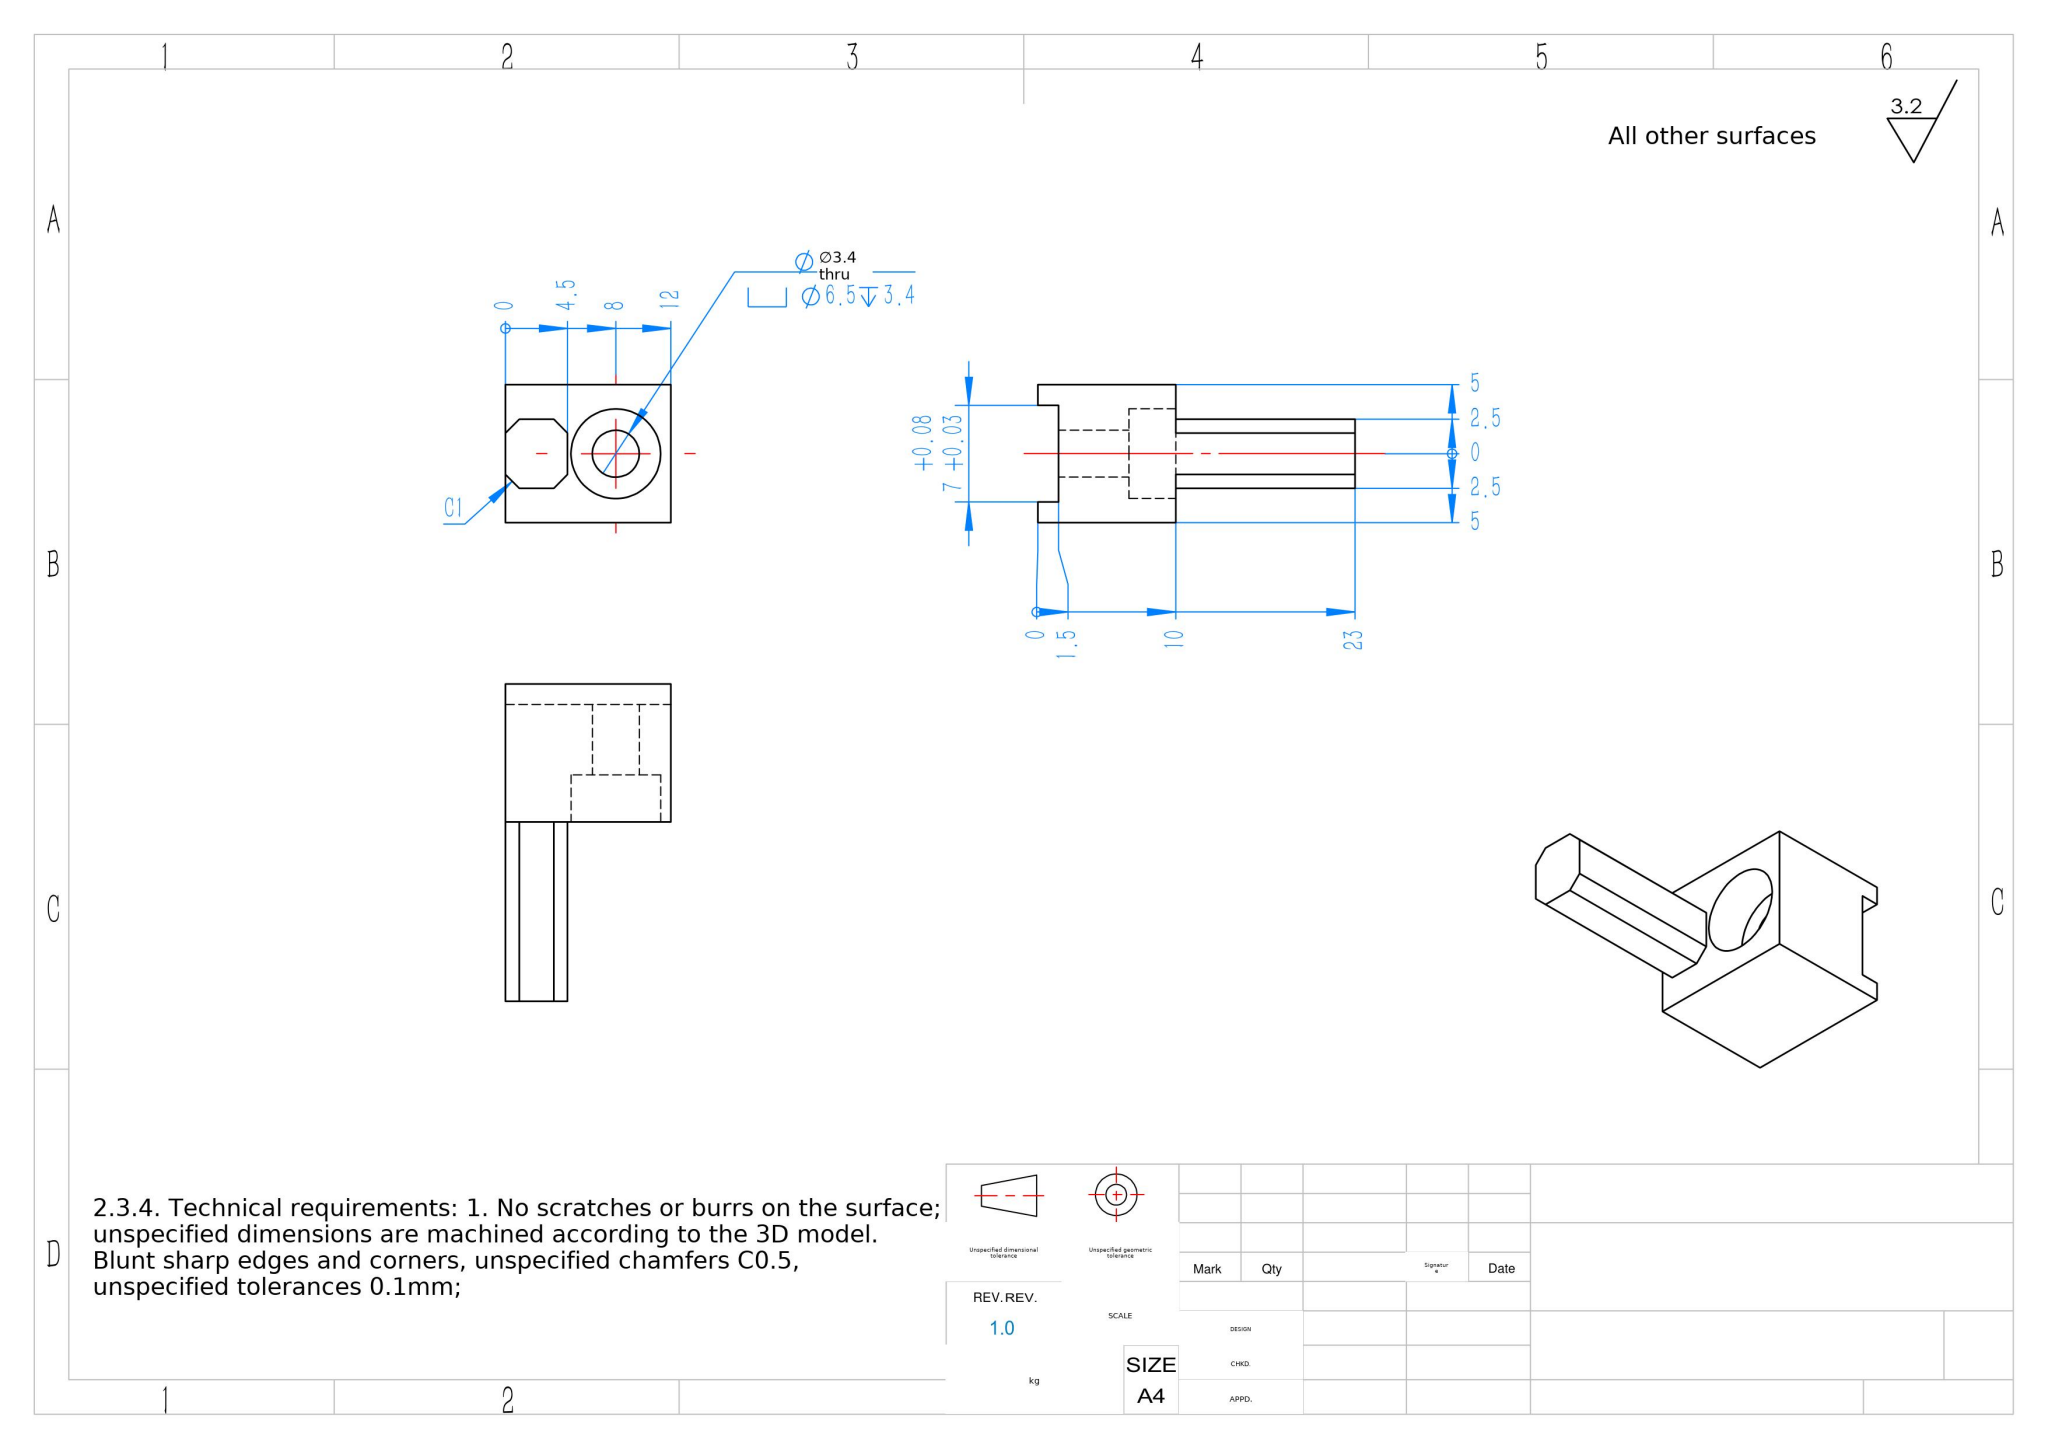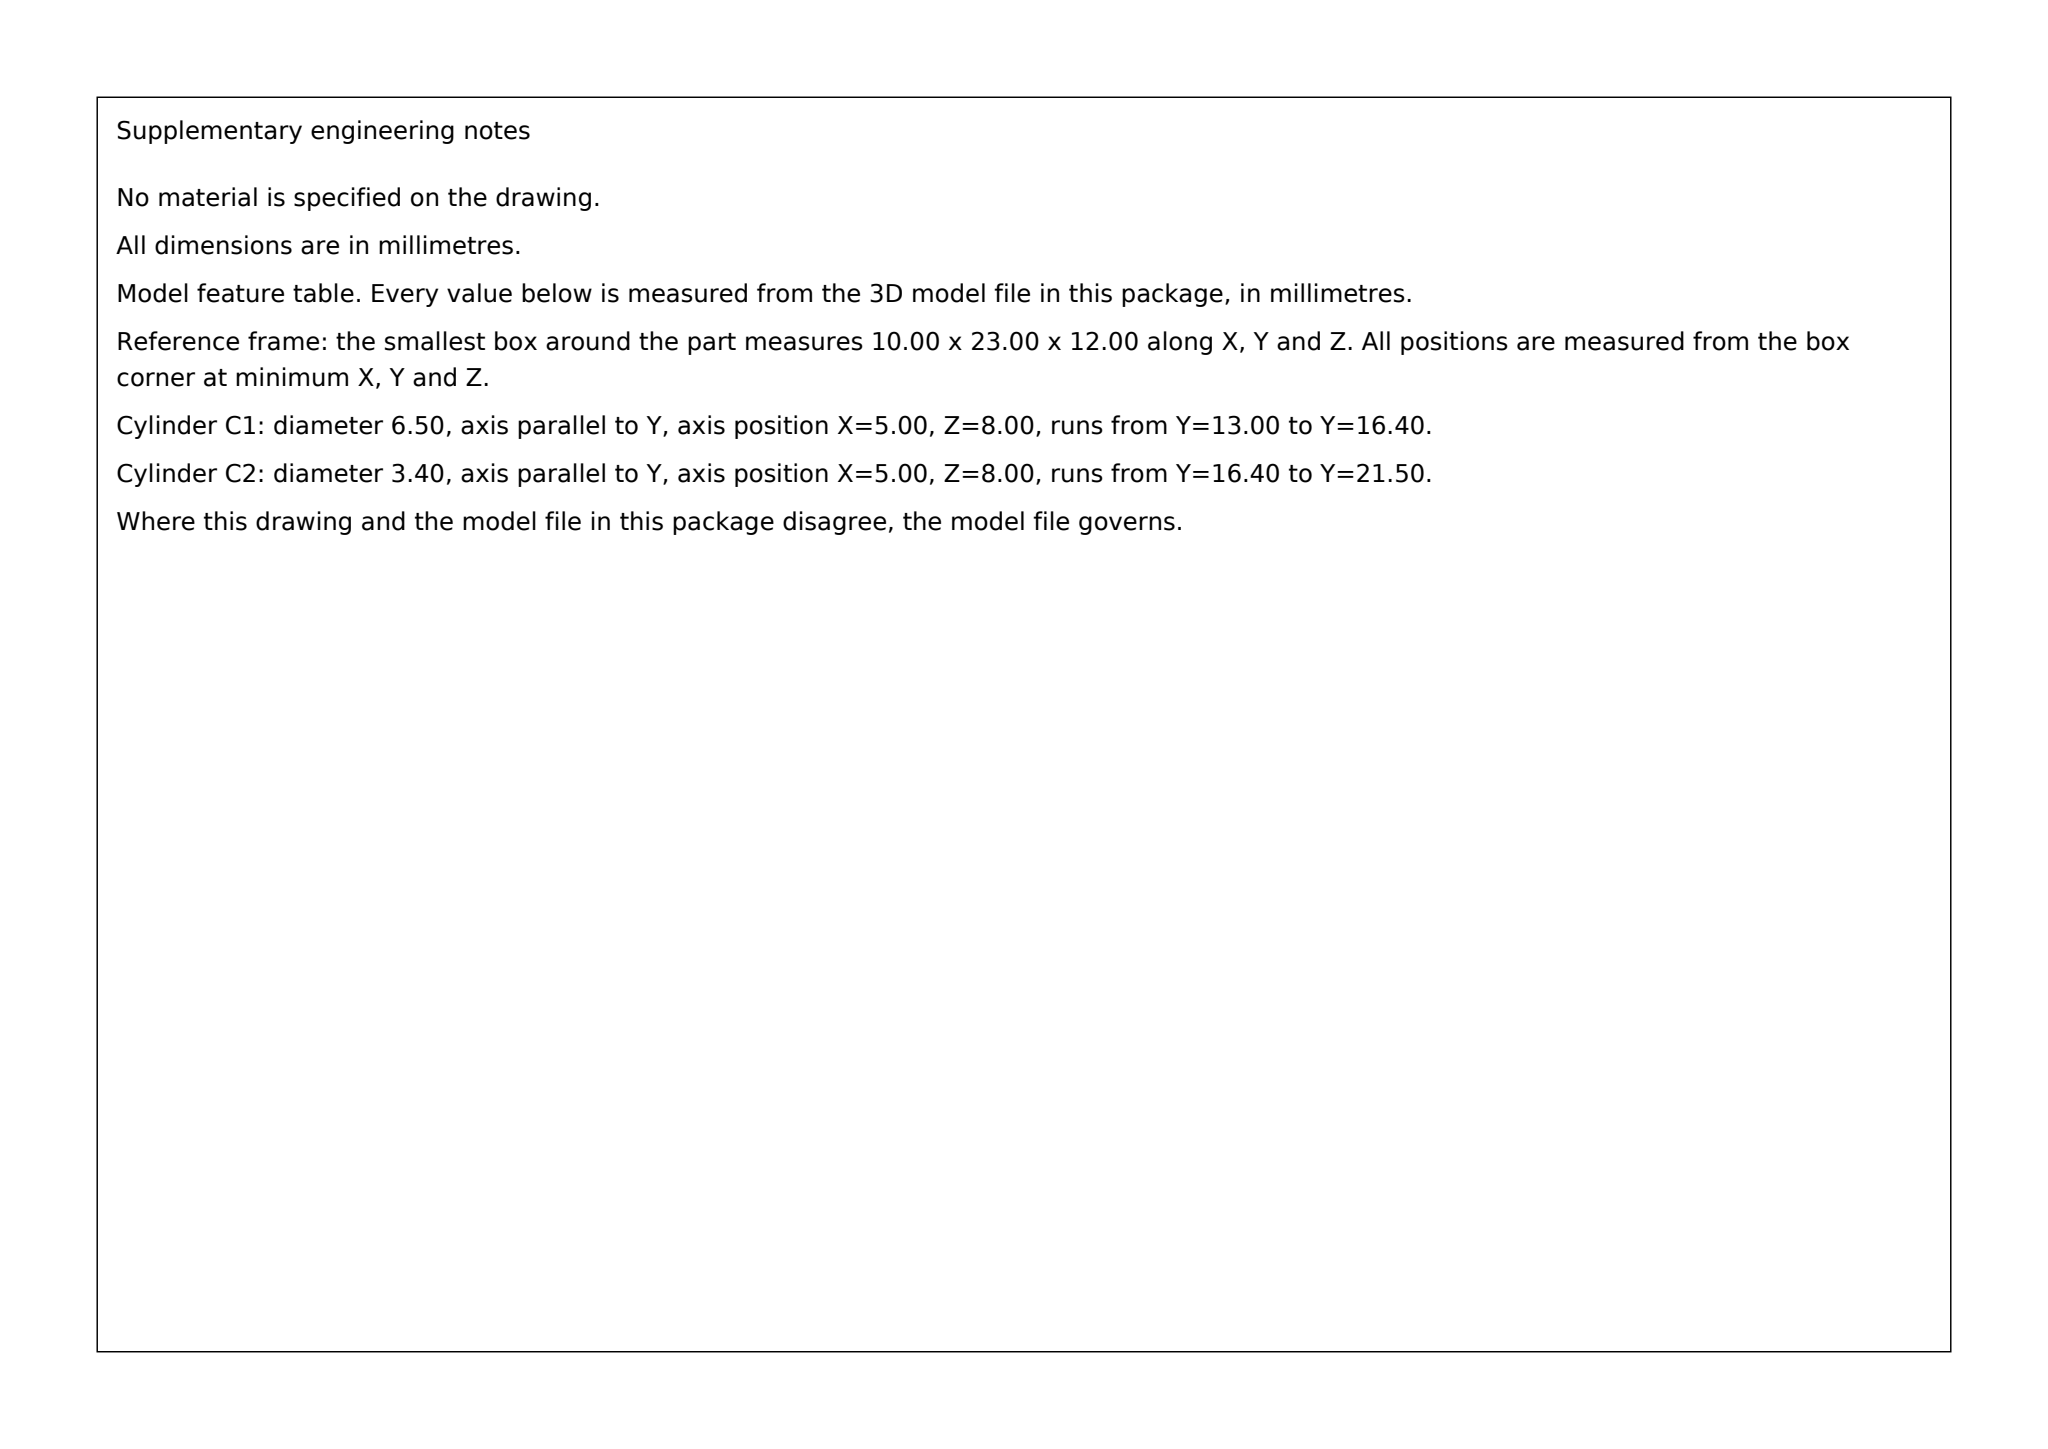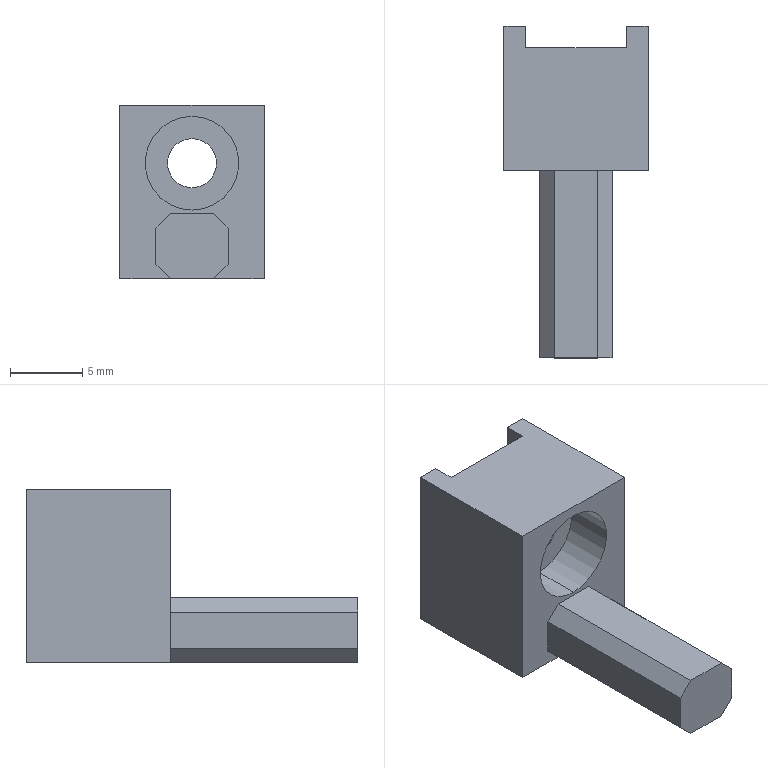Part | SolidWorks | mm | 1 solid | 23 faces | box 10 x 23 x 12 mm | volume 1181 mm3 | plane 19 | cylinder 4 | commonest cylinder face diameters 6.5 x2 3.4 x2
build123d program:
from build123d import *

# Parameters (mm, degrees)
SKETCH1_W                                       = 12
SKETCH1_H                                       = 10
BOSS_EXTRUDE1_DEPTH                             = 5
SKETCH2_W                                       = 7
SKETCH2_H                                       = 3
CUT_EXTRUDE1_DEPTH                              = 14.928
M3_HEX_SOCKET_HEAD_CAP_SCREW_CBORE1_D           = 3.4
M3_HEX_SOCKET_HEAD_CAP_SCREW_CBORE1_CBORE_D     = 6.5
M3_HEX_SOCKET_HEAD_CAP_SCREW_CBORE1_CBORE_DEPTH = 3.4
SKETCH5_W                                       = 5
SKETCH5_H                                       = 4.5
BOSS_EXTRUDE2_DEPTH                             = 13
CHAMFER1_SIZE                                   = 1


with BuildPart() as part:
    # Sketch1 → Boss-Extrude1 (new, symmetric)
    with BuildSketch(Plane(origin=(0, 0, 0), x_dir=(0, 0, -1), z_dir=(1, 0, 0))):
        Rectangle(SKETCH1_W, SKETCH1_H)
    extrude(amount=BOSS_EXTRUDE1_DEPTH, both=True)

    # Sketch2 → Cut-Extrude1 (cut, through all)
    with BuildSketch(Plane.XY.offset(6)):
        with Locations((0, 5)):
            Rectangle(SKETCH2_W, SKETCH2_H)
    extrude(amount=-CUT_EXTRUDE1_DEPTH, mode=Mode.SUBTRACT)

    # M3 Hex Socket Head Cap Screw CBORE1 (through all)
    with Locations(Plane(origin=(0, -5, 0), x_dir=(-1, 0, 0), z_dir=(0, -1, 0))):
        with Locations((0, -2)):
            CounterBoreHole(M3_HEX_SOCKET_HEAD_CAP_SCREW_CBORE1_D / 2, M3_HEX_SOCKET_HEAD_CAP_SCREW_CBORE1_CBORE_D / 2, M3_HEX_SOCKET_HEAD_CAP_SCREW_CBORE1_CBORE_DEPTH)

    # Sketch5 → Boss-Extrude2 (add)
    with BuildSketch(Plane.XZ.offset(5)):
        with Locations((0, -3.75)):
            Rectangle(SKETCH5_W, SKETCH5_H)
    extrude(amount=BOSS_EXTRUDE2_DEPTH)

    # Chamfer1
    chamfer1_edges = [part.edges().sort_by_distance(p)[0] for p in [
        (-2.5, -11.5, -1.5),
        (-2.5, -11.5, -6),
        (2.5, -11.5, -6),
        (2.5, -11.5, -1.5),
    ]]
    chamfer(chamfer1_edges, length=CHAMFER1_SIZE)


solid = part.part